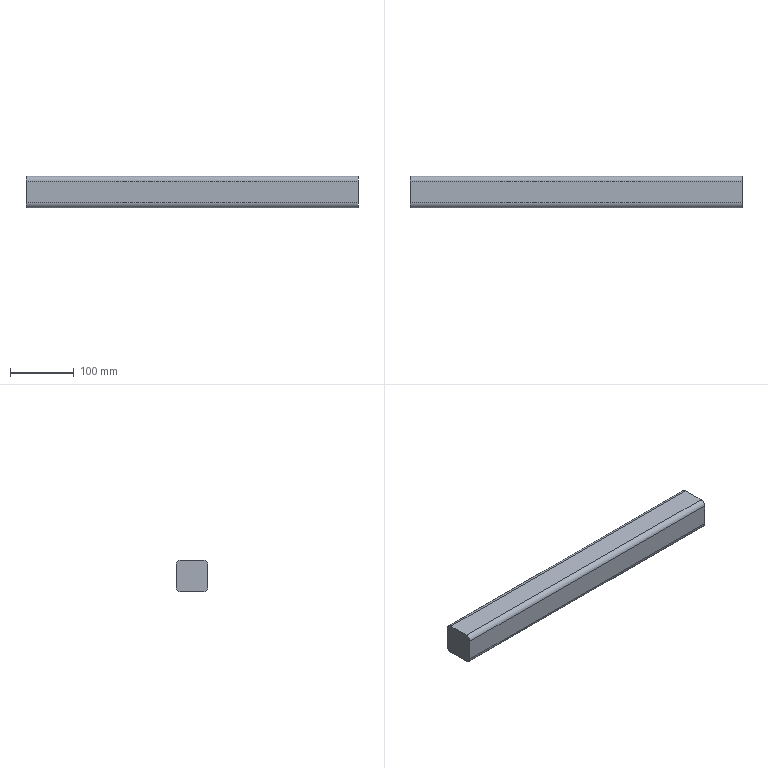Component | SolidWorks | AX00-100.1.1-1_AXFrame_A.1.1-1_AX50x50-4_square tube.1.1-3 | 1 solid | 20 faces | box 520 x 50 x 50 mm | volume 459372 mm3 | plane 12 | cylinder 8 | commonest cylinder face diameters 16 x4 6 x4 | material AISI 1035 Steel (SS)
build123d program:
from build123d import *

# Parameters (mm, degrees)
SKETCH1_W           = 50
SKETCH1_H           = 50
BOSS_EXTRUDE1_DEPTH = 260
FILLET3_R           = 8
SHELL1_T            = 5


with BuildPart() as part:
    # Sketch1 → Boss-Extrude1 (new, symmetric)
    with BuildSketch(Plane.XY):
        Rectangle(SKETCH1_W, SKETCH1_H)
    extrude(amount=BOSS_EXTRUDE1_DEPTH, both=True)

    # Fillet3
    fillet3_edges = [part.edges().sort_by_distance(p)[0] for p in [
        (25, -25, 0),
        (-25, -25, 0),
        (-25, 25, 0),
        (25, 25, 0),
    ]]
    fillet(fillet3_edges, radius=FILLET3_R)

    # Shell1 (no face opened: a closed hollow body)
    add(offset(amount=-SHELL1_T, mode=Mode.PRIVATE), mode=Mode.SUBTRACT)


solid = part.part

# Placed as in the assembly
solid = solid.moved(Location((-401.369, 1488.364, -197.5), (0, 90, 0)))